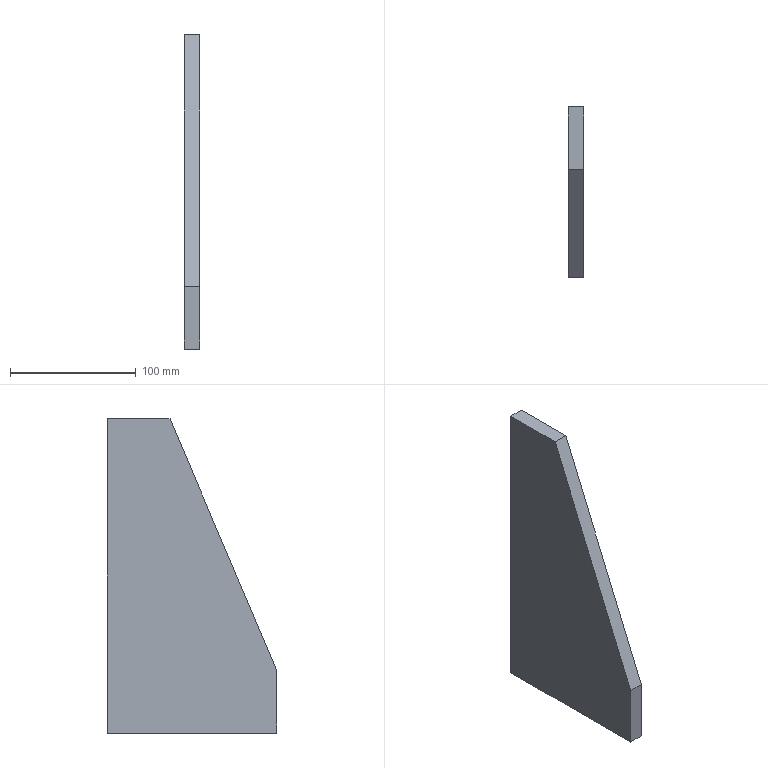Component | SolidWorks | FlangeRib2-1 | 1 solid | 7 faces | box 12 x 135 x 250 mm | volume 303000 mm3 | plane 7 | material Plain Carbon Steel
STEP:
#1=CARTESIAN_POINT('',(54.905,36.667,61.46));
#2=VERTEX_POINT('',#1);
#3=CARTESIAN_POINT('',(54.905,36.667,63.429));
#4=VERTEX_POINT('',#3);
#5=CARTESIAN_POINT('',(54.905,36.667,63.429));
#6=DIRECTION('',(-0.,0.,1.));
#7=VECTOR('',#6,39.37);
#8=LINE('',#5,#7);
#9=EDGE_CURVE('',#2,#4,#8,.T.);
#10=ORIENTED_EDGE('',*,*,#9,.F.);
#11=CARTESIAN_POINT('',(55.377,36.667,61.46));
#12=VERTEX_POINT('',#11);
#13=CARTESIAN_POINT('',(55.377,36.667,61.46));
#14=DIRECTION('',(-1.,-0.,0.));
#15=VECTOR('',#14,39.37);
#16=LINE('',#13,#15);
#17=EDGE_CURVE('',#12,#2,#16,.T.);
#18=ORIENTED_EDGE('',*,*,#17,.F.);
#19=CARTESIAN_POINT('',(55.377,36.667,63.429));
#20=VERTEX_POINT('',#19);
#21=CARTESIAN_POINT('',(55.377,36.667,63.429));
#22=DIRECTION('',(-0.,0.,1.));
#23=VECTOR('',#22,39.37);
#24=LINE('',#21,#23);
#25=EDGE_CURVE('',#12,#20,#24,.T.);
#26=ORIENTED_EDGE('',*,*,#25,.T.);
#27=CARTESIAN_POINT('',(55.377,36.667,63.429));
#28=DIRECTION('',(-1.,-0.,0.));
#29=VECTOR('',#28,39.37);
#30=LINE('',#27,#29);
#31=EDGE_CURVE('',#20,#4,#30,.T.);
#32=ORIENTED_EDGE('',*,*,#31,.T.);
#33=EDGE_LOOP('',(#10,#18,#26,#32));
#34=FACE_OUTER_BOUND('',#33,.T.);
#35=CARTESIAN_POINT('',(55.377,36.667,63.429));
#36=DIRECTION('',(0.,-1.,0.));
#37=DIRECTION('',(-1.,-0.,0.));
#38=AXIS2_PLACEMENT_3D('',#35,#36,#37);
#39=PLANE('',#38);
#40=ADVANCED_FACE('',(#34),#39,.T.);
#41=CARTESIAN_POINT('',(54.905,41.982,61.46));
#42=VERTEX_POINT('',#41);
#43=CARTESIAN_POINT('',(54.905,36.667,61.46));
#44=DIRECTION('',(0.,-1.,0.));
#45=VECTOR('',#44,39.37);
#46=LINE('',#43,#45);
#47=EDGE_CURVE('',#42,#2,#46,.T.);
#48=ORIENTED_EDGE('',*,*,#47,.F.);
#49=CARTESIAN_POINT('',(55.377,41.982,61.46));
#50=VERTEX_POINT('',#49);
#51=CARTESIAN_POINT('',(55.377,41.982,61.46));
#52=DIRECTION('',(-1.,-0.,0.));
#53=VECTOR('',#52,39.37);
#54=LINE('',#51,#53);
#55=EDGE_CURVE('',#50,#42,#54,.T.);
#56=ORIENTED_EDGE('',*,*,#55,.F.);
#57=CARTESIAN_POINT('',(55.377,36.667,61.46));
#58=DIRECTION('',(0.,-1.,0.));
#59=VECTOR('',#58,39.37);
#60=LINE('',#57,#59);
#61=EDGE_CURVE('',#50,#12,#60,.T.);
#62=ORIENTED_EDGE('',*,*,#61,.T.);
#63=ORIENTED_EDGE('',*,*,#17,.T.);
#64=EDGE_LOOP('',(#48,#56,#62,#63));
#65=FACE_OUTER_BOUND('',#64,.T.);
#66=CARTESIAN_POINT('',(55.377,36.667,61.46));
#67=DIRECTION('',(0.,-0.,-1.));
#68=DIRECTION('',(0.,-1.,0.));
#69=AXIS2_PLACEMENT_3D('',#66,#67,#68);
#70=PLANE('',#69);
#71=ADVANCED_FACE('',(#65),#70,.T.);
#72=CARTESIAN_POINT('',(54.905,41.982,71.303));
#73=VERTEX_POINT('',#72);
#74=CARTESIAN_POINT('',(54.905,41.982,61.46));
#75=DIRECTION('',(0.,-0.,-1.));
#76=VECTOR('',#75,39.37);
#77=LINE('',#74,#76);
#78=EDGE_CURVE('',#73,#42,#77,.T.);
#79=ORIENTED_EDGE('',*,*,#78,.F.);
#80=CARTESIAN_POINT('',(55.377,41.982,71.303));
#81=VERTEX_POINT('',#80);
#82=CARTESIAN_POINT('',(55.377,41.982,71.303));
#83=DIRECTION('',(-1.,-0.,0.));
#84=VECTOR('',#83,39.37);
#85=LINE('',#82,#84);
#86=EDGE_CURVE('',#81,#73,#85,.T.);
#87=ORIENTED_EDGE('',*,*,#86,.F.);
#88=CARTESIAN_POINT('',(55.377,41.982,61.46));
#89=DIRECTION('',(0.,-0.,-1.));
#90=VECTOR('',#89,39.37);
#91=LINE('',#88,#90);
#92=EDGE_CURVE('',#81,#50,#91,.T.);
#93=ORIENTED_EDGE('',*,*,#92,.T.);
#94=ORIENTED_EDGE('',*,*,#55,.T.);
#95=EDGE_LOOP('',(#79,#87,#93,#94));
#96=FACE_OUTER_BOUND('',#95,.T.);
#97=CARTESIAN_POINT('',(55.377,41.982,61.46));
#98=DIRECTION('',(-0.,1.,-0.));
#99=DIRECTION('',(0.,-0.,-1.));
#100=AXIS2_PLACEMENT_3D('',#97,#98,#99);
#101=PLANE('',#100);
#102=ADVANCED_FACE('',(#96),#101,.T.);
#103=CARTESIAN_POINT('',(54.905,40.014,71.303));
#104=VERTEX_POINT('',#103);
#105=CARTESIAN_POINT('',(54.905,41.982,71.303));
#106=DIRECTION('',(-0.,1.,-0.));
#107=VECTOR('',#106,39.37);
#108=LINE('',#105,#107);
#109=EDGE_CURVE('',#104,#73,#108,.T.);
#110=ORIENTED_EDGE('',*,*,#109,.F.);
#111=CARTESIAN_POINT('',(55.377,40.014,71.303));
#112=VERTEX_POINT('',#111);
#113=CARTESIAN_POINT('',(55.377,40.014,71.303));
#114=DIRECTION('',(-1.,-0.,0.));
#115=VECTOR('',#114,39.37);
#116=LINE('',#113,#115);
#117=EDGE_CURVE('',#112,#104,#116,.T.);
#118=ORIENTED_EDGE('',*,*,#117,.F.);
#119=CARTESIAN_POINT('',(55.377,41.982,71.303));
#120=DIRECTION('',(-0.,1.,-0.));
#121=VECTOR('',#120,39.37);
#122=LINE('',#119,#121);
#123=EDGE_CURVE('',#112,#81,#122,.T.);
#124=ORIENTED_EDGE('',*,*,#123,.T.);
#125=ORIENTED_EDGE('',*,*,#86,.T.);
#126=EDGE_LOOP('',(#110,#118,#124,#125));
#127=FACE_OUTER_BOUND('',#126,.T.);
#128=CARTESIAN_POINT('',(55.377,41.982,71.303));
#129=DIRECTION('',(-0.,0.,1.));
#130=DIRECTION('',(-0.,1.,-0.));
#131=AXIS2_PLACEMENT_3D('',#128,#129,#130);
#132=PLANE('',#131);
#133=ADVANCED_FACE('',(#127),#132,.T.);
#134=CARTESIAN_POINT('',(54.905,40.014,71.303));
#135=DIRECTION('',(-0.,0.3911,0.9203));
#136=VECTOR('',#135,39.37);
#137=LINE('',#134,#136);
#138=EDGE_CURVE('',#4,#104,#137,.T.);
#139=ORIENTED_EDGE('',*,*,#138,.F.);
#140=ORIENTED_EDGE('',*,*,#31,.F.);
#141=CARTESIAN_POINT('',(55.377,40.014,71.303));
#142=DIRECTION('',(-0.,0.3911,0.9203));
#143=VECTOR('',#142,39.37);
#144=LINE('',#141,#143);
#145=EDGE_CURVE('',#20,#112,#144,.T.);
#146=ORIENTED_EDGE('',*,*,#145,.T.);
#147=ORIENTED_EDGE('',*,*,#117,.T.);
#148=EDGE_LOOP('',(#139,#140,#146,#147));
#149=FACE_OUTER_BOUND('',#148,.T.);
#150=CARTESIAN_POINT('',(55.377,40.014,71.303));
#151=DIRECTION('',(0.,-0.9203,0.3911));
#152=DIRECTION('',(-0.,0.3911,0.9203));
#153=AXIS2_PLACEMENT_3D('',#150,#151,#152);
#154=PLANE('',#153);
#155=ADVANCED_FACE('',(#149),#154,.T.);
#156=ORIENTED_EDGE('',*,*,#25,.F.);
#157=ORIENTED_EDGE('',*,*,#61,.F.);
#158=ORIENTED_EDGE('',*,*,#92,.F.);
#159=ORIENTED_EDGE('',*,*,#123,.F.);
#160=ORIENTED_EDGE('',*,*,#145,.F.);
#161=EDGE_LOOP('',(#156,#157,#158,#159,#160));
#162=FACE_OUTER_BOUND('',#161,.T.);
#163=CARTESIAN_POINT('',(55.377,36.667,61.46));
#164=DIRECTION('',(1.,0.,0.));
#165=DIRECTION('',(0.,-1.,0.));
#166=AXIS2_PLACEMENT_3D('',#163,#164,#165);
#167=PLANE('',#166);
#168=ADVANCED_FACE('',(#162),#167,.T.);
#169=ORIENTED_EDGE('',*,*,#9,.T.);
#170=ORIENTED_EDGE('',*,*,#138,.T.);
#171=ORIENTED_EDGE('',*,*,#109,.T.);
#172=ORIENTED_EDGE('',*,*,#78,.T.);
#173=ORIENTED_EDGE('',*,*,#47,.T.);
#174=EDGE_LOOP('',(#169,#170,#171,#172,#173));
#175=FACE_OUTER_BOUND('',#174,.T.);
#176=CARTESIAN_POINT('',(54.905,36.667,61.46));
#177=DIRECTION('',(1.,0.,0.));
#178=DIRECTION('',(0.,-1.,0.));
#179=AXIS2_PLACEMENT_3D('',#176,#177,#178);
#180=PLANE('',#179);
#181=ADVANCED_FACE('',(#175),#180,.F.);
#182=CLOSED_SHELL('',(#40,#71,#102,#133,#155,#168,#181));
#183=MANIFOLD_SOLID_BREP('',#182);
#184=CARTESIAN_POINT('',(0.,0.,0.));
#185=DIRECTION('',(0.,0.,1.));
#186=DIRECTION('',(1.,0.,0.));
#187=AXIS2_PLACEMENT_3D('',#184,#185,#186);
#188=(LENGTH_UNIT()NAMED_UNIT(*)SI_UNIT($,.METRE.));
#189=LENGTH_MEASURE_WITH_UNIT(LENGTH_MEASURE(0.0254),#188);
#190=DIMENSIONAL_EXPONENTS(1.,0.,0.,0.,0.,0.,0.);
#191=(CONVERSION_BASED_UNIT('',#189)LENGTH_UNIT()NAMED_UNIT(#190));
#192=UNCERTAINTY_MEASURE_WITH_UNIT(LENGTH_MEASURE(0.00001),#191,'','');
#193=(NAMED_UNIT(*)PLANE_ANGLE_UNIT()SI_UNIT($,.RADIAN.));
#194=(NAMED_UNIT(*)SI_UNIT($,.STERADIAN.)SOLID_ANGLE_UNIT());
#195=(GEOMETRIC_REPRESENTATION_CONTEXT(3)GLOBAL_UNCERTAINTY_ASSIGNED_CONTEXT((#192))GLOBAL_UNIT_ASSIGNED_CONTEXT((#191,#193,#194))REPRESENTATION_CONTEXT('',''));
#196=ADVANCED_BREP_SHAPE_REPRESENTATION('',(#183,#187),#195);
#197=COLOUR_RGB('',0.7922,0.8196,0.9333);
#198=FILL_AREA_STYLE_COLOUR('',#197);
#199=FILL_AREA_STYLE('',(#198));
#200=SURFACE_STYLE_FILL_AREA(#199);
#201=SURFACE_SIDE_STYLE('',(#200));
#202=SURFACE_STYLE_USAGE(.BOTH.,#201);
#203=PRESENTATION_STYLE_ASSIGNMENT((#202));
#204=STYLED_ITEM('',(#203),#183);
#205=(LENGTH_UNIT()NAMED_UNIT(*)SI_UNIT($,.METRE.));
#206=LENGTH_MEASURE_WITH_UNIT(LENGTH_MEASURE(0.0254),#205);
#207=DIMENSIONAL_EXPONENTS(1.,0.,0.,0.,0.,0.,0.);
#208=(CONVERSION_BASED_UNIT('',#206)LENGTH_UNIT()NAMED_UNIT(#207));
#209=UNCERTAINTY_MEASURE_WITH_UNIT(LENGTH_MEASURE(0.00001),#208,'','');
#210=(NAMED_UNIT(*)PLANE_ANGLE_UNIT()SI_UNIT($,.RADIAN.));
#211=(NAMED_UNIT(*)SI_UNIT($,.STERADIAN.)SOLID_ANGLE_UNIT());
#212=(GEOMETRIC_REPRESENTATION_CONTEXT(3)GLOBAL_UNCERTAINTY_ASSIGNED_CONTEXT((#209))GLOBAL_UNIT_ASSIGNED_CONTEXT((#208,#210,#211))REPRESENTATION_CONTEXT('',''));
#213=MECHANICAL_DESIGN_GEOMETRIC_PRESENTATION_REPRESENTATION('',(#204),#212);
#214=PRESENTATION_LAYER_ASSIGNMENT('','',(#204));